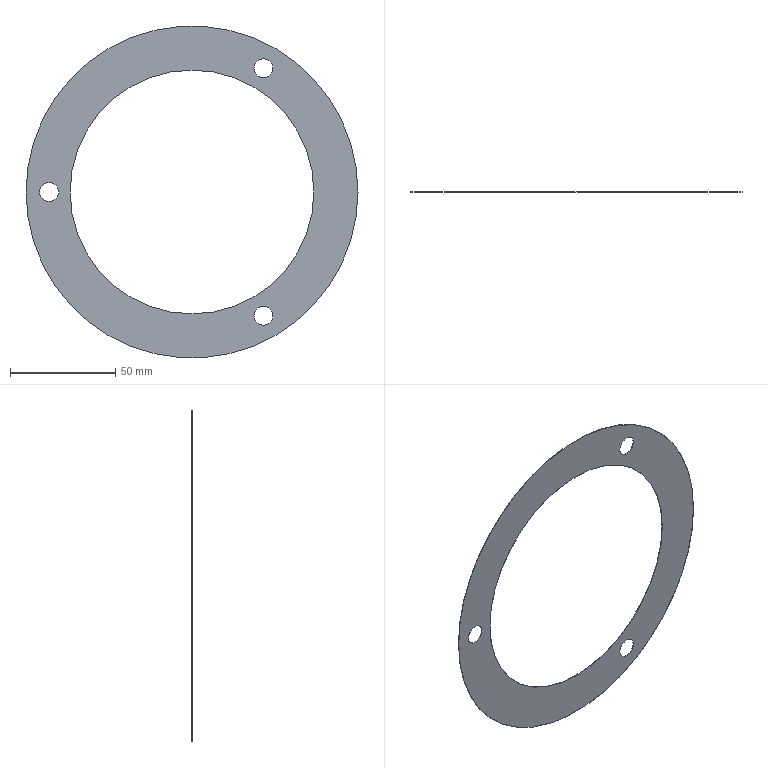Component | SolidWorks | 22-1 | 1 solid | 12 faces | box 158 x 0.2 x 158 mm | volume 1770 mm3 | cylinder 10 | plane 2 | commonest cylinder face diameters 9 x6 116 x2 158 x2
build123d program:
from build123d import *

# Parameters (mm, degrees)
SKETCH1_R           = 79
SKETCH1_R_2         = 58
SKETCH1_R_3         = 4.5
BOSS_EXTRUDE1_DEPTH = 0.2


with BuildPart() as part:
    # Sketch1 → Boss-Extrude1 (new body)
    with BuildSketch(Plane(origin=(0, 0, 0), x_dir=(1, 0, 0), z_dir=(0, 1, 0))):
        with Locations(Location((0, 0, 0), (0, 0, 270))):
            Circle(SKETCH1_R)
        with Locations(Location((0, 0, 0), (0, 0, 270))):
            Circle(SKETCH1_R_2, mode=Mode.SUBTRACT)
        with Locations(Location((0, -68, 0), (0, 0, 270))):
            Circle(SKETCH1_R_3, mode=Mode.SUBTRACT)
        with Locations(Location((-58.89, 34, 0), (0, 0, 270))):
            Circle(SKETCH1_R_3, mode=Mode.SUBTRACT)
        with Locations(Location((58.89, 34, 0), (0, 0, 270))):
            Circle(SKETCH1_R_3, mode=Mode.SUBTRACT)
    extrude(amount=BOSS_EXTRUDE1_DEPTH)


solid = part.part

# Placed as in the assembly
solid = solid.moved(Location((0, 15, 0), (0, -90, 0)))
STEP:
#1=COLOUR_RGB('',0.7922,0.8196,0.9333);
#2=FILL_AREA_STYLE_COLOUR('',#1);
#3=FILL_AREA_STYLE('',(#2));
#4=SURFACE_STYLE_FILL_AREA(#3);
#5=SURFACE_SIDE_STYLE('',(#4));
#6=SURFACE_STYLE_USAGE(.BOTH.,#5);
#7=PRESENTATION_STYLE_ASSIGNMENT((#6));
#8=CARTESIAN_POINT('',(1.516,0.5984,2.318));
#9=VERTEX_POINT('',#8);
#10=CARTESIAN_POINT('',(1.161,0.5984,2.318));
#11=VERTEX_POINT('',#10);
#12=CARTESIAN_POINT('',(1.339,0.5984,2.318));
#13=DIRECTION('',(-0.,1.,0.));
#14=DIRECTION('',(-1.,0.,0.));
#15=AXIS2_PLACEMENT_3D('',#12,#13,#14);
#16=CIRCLE('',#15,0.1772);
#17=EDGE_CURVE('',#9,#11,#16,.T.);
#18=ORIENTED_EDGE('',*,*,#17,.T.);
#19=CARTESIAN_POINT('',(1.161,0.5906,2.318));
#20=VERTEX_POINT('',#19);
#21=CARTESIAN_POINT('',(1.161,0.5984,2.318));
#22=DIRECTION('',(0.,-1.,-0.));
#23=VECTOR('',#22,39.37);
#24=LINE('',#21,#23);
#25=EDGE_CURVE('',#11,#20,#24,.T.);
#26=ORIENTED_EDGE('',*,*,#25,.T.);
#27=CARTESIAN_POINT('',(1.516,0.5906,2.318));
#28=VERTEX_POINT('',#27);
#29=CARTESIAN_POINT('',(1.339,0.5906,2.318));
#30=DIRECTION('',(-0.,1.,0.));
#31=DIRECTION('',(-1.,0.,0.));
#32=AXIS2_PLACEMENT_3D('',#29,#30,#31);
#33=CIRCLE('',#32,0.1772);
#34=EDGE_CURVE('',#28,#20,#33,.T.);
#35=ORIENTED_EDGE('',*,*,#34,.F.);
#36=CARTESIAN_POINT('',(1.516,0.5984,2.318));
#37=DIRECTION('',(0.,-1.,-0.));
#38=VECTOR('',#37,39.37);
#39=LINE('',#36,#38);
#40=EDGE_CURVE('',#9,#28,#39,.T.);
#41=ORIENTED_EDGE('',*,*,#40,.F.);
#42=EDGE_LOOP('',(#18,#26,#35,#41));
#43=FACE_OUTER_BOUND('',#42,.T.);
#44=CARTESIAN_POINT('',(1.339,0.5984,2.318));
#45=DIRECTION('',(0.,-1.,-0.));
#46=DIRECTION('',(1.,0.,-0.));
#47=AXIS2_PLACEMENT_3D('',#44,#45,#46);
#48=CYLINDRICAL_SURFACE('',#47,0.1772);
#49=ADVANCED_FACE('',(#43),#48,.F.);
#50=CARTESIAN_POINT('',(1.516,0.5984,-2.318));
#51=VERTEX_POINT('',#50);
#52=CARTESIAN_POINT('',(1.161,0.5984,-2.318));
#53=VERTEX_POINT('',#52);
#54=CARTESIAN_POINT('',(1.339,0.5984,-2.318));
#55=DIRECTION('',(-0.,1.,0.));
#56=DIRECTION('',(-1.,0.,0.));
#57=AXIS2_PLACEMENT_3D('',#54,#55,#56);
#58=CIRCLE('',#57,0.1772);
#59=EDGE_CURVE('',#51,#53,#58,.T.);
#60=ORIENTED_EDGE('',*,*,#59,.T.);
#61=CARTESIAN_POINT('',(1.161,0.5906,-2.318));
#62=VERTEX_POINT('',#61);
#63=CARTESIAN_POINT('',(1.161,0.5984,-2.318));
#64=DIRECTION('',(0.,-1.,-0.));
#65=VECTOR('',#64,39.37);
#66=LINE('',#63,#65);
#67=EDGE_CURVE('',#53,#62,#66,.T.);
#68=ORIENTED_EDGE('',*,*,#67,.T.);
#69=CARTESIAN_POINT('',(1.516,0.5906,-2.318));
#70=VERTEX_POINT('',#69);
#71=CARTESIAN_POINT('',(1.339,0.5906,-2.318));
#72=DIRECTION('',(-0.,1.,0.));
#73=DIRECTION('',(-1.,0.,0.));
#74=AXIS2_PLACEMENT_3D('',#71,#72,#73);
#75=CIRCLE('',#74,0.1772);
#76=EDGE_CURVE('',#70,#62,#75,.T.);
#77=ORIENTED_EDGE('',*,*,#76,.F.);
#78=CARTESIAN_POINT('',(1.516,0.5984,-2.318));
#79=DIRECTION('',(0.,-1.,-0.));
#80=VECTOR('',#79,39.37);
#81=LINE('',#78,#80);
#82=EDGE_CURVE('',#51,#70,#81,.T.);
#83=ORIENTED_EDGE('',*,*,#82,.F.);
#84=EDGE_LOOP('',(#60,#68,#77,#83));
#85=FACE_OUTER_BOUND('',#84,.T.);
#86=CARTESIAN_POINT('',(1.339,0.5984,-2.318));
#87=DIRECTION('',(0.,-1.,-0.));
#88=DIRECTION('',(1.,0.,-0.));
#89=AXIS2_PLACEMENT_3D('',#86,#87,#88);
#90=CYLINDRICAL_SURFACE('',#89,0.1772);
#91=ADVANCED_FACE('',(#85),#90,.F.);
#92=CARTESIAN_POINT('',(-2.5,0.5984,0.));
#93=VERTEX_POINT('',#92);
#94=CARTESIAN_POINT('',(-2.854,0.5984,0.));
#95=VERTEX_POINT('',#94);
#96=CARTESIAN_POINT('',(-2.677,0.5984,0.));
#97=DIRECTION('',(-0.,1.,0.));
#98=DIRECTION('',(-1.,0.,0.));
#99=AXIS2_PLACEMENT_3D('',#96,#97,#98);
#100=CIRCLE('',#99,0.1772);
#101=EDGE_CURVE('',#93,#95,#100,.T.);
#102=ORIENTED_EDGE('',*,*,#101,.T.);
#103=CARTESIAN_POINT('',(-2.854,0.5906,0.));
#104=VERTEX_POINT('',#103);
#105=CARTESIAN_POINT('',(-2.854,0.5984,0.));
#106=DIRECTION('',(0.,-1.,-0.));
#107=VECTOR('',#106,39.37);
#108=LINE('',#105,#107);
#109=EDGE_CURVE('',#95,#104,#108,.T.);
#110=ORIENTED_EDGE('',*,*,#109,.T.);
#111=CARTESIAN_POINT('',(-2.5,0.5906,0.));
#112=VERTEX_POINT('',#111);
#113=CARTESIAN_POINT('',(-2.677,0.5906,0.));
#114=DIRECTION('',(-0.,1.,0.));
#115=DIRECTION('',(-1.,0.,0.));
#116=AXIS2_PLACEMENT_3D('',#113,#114,#115);
#117=CIRCLE('',#116,0.1772);
#118=EDGE_CURVE('',#112,#104,#117,.T.);
#119=ORIENTED_EDGE('',*,*,#118,.F.);
#120=CARTESIAN_POINT('',(-2.5,0.5984,0.));
#121=DIRECTION('',(0.,-1.,-0.));
#122=VECTOR('',#121,39.37);
#123=LINE('',#120,#122);
#124=EDGE_CURVE('',#93,#112,#123,.T.);
#125=ORIENTED_EDGE('',*,*,#124,.F.);
#126=EDGE_LOOP('',(#102,#110,#119,#125));
#127=FACE_OUTER_BOUND('',#126,.T.);
#128=CARTESIAN_POINT('',(-2.677,0.5984,0.));
#129=DIRECTION('',(0.,-1.,-0.));
#130=DIRECTION('',(1.,0.,-0.));
#131=AXIS2_PLACEMENT_3D('',#128,#129,#130);
#132=CYLINDRICAL_SURFACE('',#131,0.1772);
#133=ADVANCED_FACE('',(#127),#132,.F.);
#134=CARTESIAN_POINT('',(2.283,0.5984,-0.));
#135=VERTEX_POINT('',#134);
#136=CARTESIAN_POINT('',(-2.283,0.5984,0.));
#137=VERTEX_POINT('',#136);
#138=CARTESIAN_POINT('',(0.,0.5984,0.));
#139=DIRECTION('',(-0.,1.,0.));
#140=DIRECTION('',(-1.,-0.,0.));
#141=AXIS2_PLACEMENT_3D('',#138,#139,#140);
#142=CIRCLE('',#141,2.283);
#143=EDGE_CURVE('',#135,#137,#142,.T.);
#144=ORIENTED_EDGE('',*,*,#143,.T.);
#145=CARTESIAN_POINT('',(-2.283,0.5906,0.));
#146=VERTEX_POINT('',#145);
#147=CARTESIAN_POINT('',(-2.283,0.5984,0.));
#148=DIRECTION('',(0.,-1.,-0.));
#149=VECTOR('',#148,39.37);
#150=LINE('',#147,#149);
#151=EDGE_CURVE('',#137,#146,#150,.T.);
#152=ORIENTED_EDGE('',*,*,#151,.T.);
#153=CARTESIAN_POINT('',(2.283,0.5906,-0.));
#154=VERTEX_POINT('',#153);
#155=CARTESIAN_POINT('',(0.,0.5906,0.));
#156=DIRECTION('',(-0.,1.,0.));
#157=DIRECTION('',(-1.,-0.,0.));
#158=AXIS2_PLACEMENT_3D('',#155,#156,#157);
#159=CIRCLE('',#158,2.283);
#160=EDGE_CURVE('',#154,#146,#159,.T.);
#161=ORIENTED_EDGE('',*,*,#160,.F.);
#162=CARTESIAN_POINT('',(2.283,0.5984,-0.));
#163=DIRECTION('',(0.,-1.,-0.));
#164=VECTOR('',#163,39.37);
#165=LINE('',#162,#164);
#166=EDGE_CURVE('',#135,#154,#165,.T.);
#167=ORIENTED_EDGE('',*,*,#166,.F.);
#168=EDGE_LOOP('',(#144,#152,#161,#167));
#169=FACE_OUTER_BOUND('',#168,.T.);
#170=CARTESIAN_POINT('',(0.,0.5984,0.));
#171=DIRECTION('',(0.,-1.,-0.));
#172=DIRECTION('',(1.,0.,-0.));
#173=AXIS2_PLACEMENT_3D('',#170,#171,#172);
#174=CYLINDRICAL_SURFACE('',#173,2.283);
#175=ADVANCED_FACE('',(#169),#174,.F.);
#176=CARTESIAN_POINT('',(-3.11,0.5984,0.));
#177=VERTEX_POINT('',#176);
#178=CARTESIAN_POINT('',(3.11,0.5984,-0.));
#179=VERTEX_POINT('',#178);
#180=CARTESIAN_POINT('',(0.,0.5984,0.));
#181=DIRECTION('',(-0.,1.,0.));
#182=DIRECTION('',(-1.,-0.,0.));
#183=AXIS2_PLACEMENT_3D('',#180,#181,#182);
#184=CIRCLE('',#183,3.11);
#185=EDGE_CURVE('',#177,#179,#184,.T.);
#186=ORIENTED_EDGE('',*,*,#185,.F.);
#187=CARTESIAN_POINT('',(-3.11,0.5906,0.));
#188=VERTEX_POINT('',#187);
#189=CARTESIAN_POINT('',(-3.11,0.5984,0.));
#190=DIRECTION('',(0.,-1.,-0.));
#191=VECTOR('',#190,39.37);
#192=LINE('',#189,#191);
#193=EDGE_CURVE('',#177,#188,#192,.T.);
#194=ORIENTED_EDGE('',*,*,#193,.T.);
#195=CARTESIAN_POINT('',(3.11,0.5906,-0.));
#196=VERTEX_POINT('',#195);
#197=CARTESIAN_POINT('',(0.,0.5906,0.));
#198=DIRECTION('',(-0.,1.,0.));
#199=DIRECTION('',(-1.,-0.,0.));
#200=AXIS2_PLACEMENT_3D('',#197,#198,#199);
#201=CIRCLE('',#200,3.11);
#202=EDGE_CURVE('',#188,#196,#201,.T.);
#203=ORIENTED_EDGE('',*,*,#202,.T.);
#204=CARTESIAN_POINT('',(3.11,0.5984,-0.));
#205=DIRECTION('',(0.,-1.,-0.));
#206=VECTOR('',#205,39.37);
#207=LINE('',#204,#206);
#208=EDGE_CURVE('',#179,#196,#207,.T.);
#209=ORIENTED_EDGE('',*,*,#208,.F.);
#210=EDGE_LOOP('',(#186,#194,#203,#209));
#211=FACE_OUTER_BOUND('',#210,.T.);
#212=CARTESIAN_POINT('',(0.,0.5984,0.));
#213=DIRECTION('',(0.,-1.,-0.));
#214=DIRECTION('',(1.,0.,-0.));
#215=AXIS2_PLACEMENT_3D('',#212,#213,#214);
#216=CYLINDRICAL_SURFACE('',#215,3.11);
#217=ADVANCED_FACE('',(#211),#216,.T.);
#218=ORIENTED_EDGE('',*,*,#59,.F.);
#219=CARTESIAN_POINT('',(1.339,0.5984,-2.318));
#220=DIRECTION('',(-0.,1.,0.));
#221=DIRECTION('',(-1.,0.,0.));
#222=AXIS2_PLACEMENT_3D('',#219,#220,#221);
#223=CIRCLE('',#222,0.1772);
#224=EDGE_CURVE('',#53,#51,#223,.T.);
#225=ORIENTED_EDGE('',*,*,#224,.F.);
#226=EDGE_LOOP('',(#218,#225));
#227=FACE_BOUND('',#226,.T.);
#228=ORIENTED_EDGE('',*,*,#143,.F.);
#229=CARTESIAN_POINT('',(0.,0.5984,0.));
#230=DIRECTION('',(-0.,1.,0.));
#231=DIRECTION('',(-1.,-0.,0.));
#232=AXIS2_PLACEMENT_3D('',#229,#230,#231);
#233=CIRCLE('',#232,2.283);
#234=EDGE_CURVE('',#137,#135,#233,.T.);
#235=ORIENTED_EDGE('',*,*,#234,.F.);
#236=EDGE_LOOP('',(#228,#235));
#237=FACE_BOUND('',#236,.T.);
#238=CARTESIAN_POINT('',(0.,0.5984,0.));
#239=DIRECTION('',(-0.,1.,0.));
#240=DIRECTION('',(-1.,-0.,0.));
#241=AXIS2_PLACEMENT_3D('',#238,#239,#240);
#242=CIRCLE('',#241,3.11);
#243=EDGE_CURVE('',#179,#177,#242,.T.);
#244=ORIENTED_EDGE('',*,*,#243,.T.);
#245=ORIENTED_EDGE('',*,*,#185,.T.);
#246=EDGE_LOOP('',(#244,#245));
#247=FACE_OUTER_BOUND('',#246,.T.);
#248=ORIENTED_EDGE('',*,*,#101,.F.);
#249=CARTESIAN_POINT('',(-2.677,0.5984,0.));
#250=DIRECTION('',(-0.,1.,0.));
#251=DIRECTION('',(-1.,0.,0.));
#252=AXIS2_PLACEMENT_3D('',#249,#250,#251);
#253=CIRCLE('',#252,0.1772);
#254=EDGE_CURVE('',#95,#93,#253,.T.);
#255=ORIENTED_EDGE('',*,*,#254,.F.);
#256=EDGE_LOOP('',(#248,#255));
#257=FACE_BOUND('',#256,.T.);
#258=ORIENTED_EDGE('',*,*,#17,.F.);
#259=CARTESIAN_POINT('',(1.339,0.5984,2.318));
#260=DIRECTION('',(-0.,1.,0.));
#261=DIRECTION('',(-1.,0.,0.));
#262=AXIS2_PLACEMENT_3D('',#259,#260,#261);
#263=CIRCLE('',#262,0.1772);
#264=EDGE_CURVE('',#11,#9,#263,.T.);
#265=ORIENTED_EDGE('',*,*,#264,.F.);
#266=EDGE_LOOP('',(#258,#265));
#267=FACE_BOUND('',#266,.T.);
#268=CARTESIAN_POINT('',(0.,0.5984,0.));
#269=DIRECTION('',(-0.,1.,0.));
#270=DIRECTION('',(-1.,-0.,0.));
#271=AXIS2_PLACEMENT_3D('',#268,#269,#270);
#272=PLANE('',#271);
#273=ADVANCED_FACE('',(#227,#237,#247,#257,#267),#272,.T.);
#274=CARTESIAN_POINT('',(0.,0.5906,0.));
#275=DIRECTION('',(-0.,1.,0.));
#276=DIRECTION('',(-1.,-0.,0.));
#277=AXIS2_PLACEMENT_3D('',#274,#275,#276);
#278=CIRCLE('',#277,3.11);
#279=EDGE_CURVE('',#196,#188,#278,.T.);
#280=ORIENTED_EDGE('',*,*,#279,.F.);
#281=ORIENTED_EDGE('',*,*,#202,.F.);
#282=EDGE_LOOP('',(#280,#281));
#283=FACE_OUTER_BOUND('',#282,.T.);
#284=ORIENTED_EDGE('',*,*,#160,.T.);
#285=CARTESIAN_POINT('',(0.,0.5906,0.));
#286=DIRECTION('',(-0.,1.,0.));
#287=DIRECTION('',(-1.,-0.,0.));
#288=AXIS2_PLACEMENT_3D('',#285,#286,#287);
#289=CIRCLE('',#288,2.283);
#290=EDGE_CURVE('',#146,#154,#289,.T.);
#291=ORIENTED_EDGE('',*,*,#290,.T.);
#292=EDGE_LOOP('',(#284,#291));
#293=FACE_BOUND('',#292,.T.);
#294=ORIENTED_EDGE('',*,*,#118,.T.);
#295=CARTESIAN_POINT('',(-2.677,0.5906,0.));
#296=DIRECTION('',(-0.,1.,0.));
#297=DIRECTION('',(-1.,0.,0.));
#298=AXIS2_PLACEMENT_3D('',#295,#296,#297);
#299=CIRCLE('',#298,0.1772);
#300=EDGE_CURVE('',#104,#112,#299,.T.);
#301=ORIENTED_EDGE('',*,*,#300,.T.);
#302=EDGE_LOOP('',(#294,#301));
#303=FACE_BOUND('',#302,.T.);
#304=ORIENTED_EDGE('',*,*,#76,.T.);
#305=CARTESIAN_POINT('',(1.339,0.5906,-2.318));
#306=DIRECTION('',(-0.,1.,0.));
#307=DIRECTION('',(-1.,0.,0.));
#308=AXIS2_PLACEMENT_3D('',#305,#306,#307);
#309=CIRCLE('',#308,0.1772);
#310=EDGE_CURVE('',#62,#70,#309,.T.);
#311=ORIENTED_EDGE('',*,*,#310,.T.);
#312=EDGE_LOOP('',(#304,#311));
#313=FACE_BOUND('',#312,.T.);
#314=ORIENTED_EDGE('',*,*,#34,.T.);
#315=CARTESIAN_POINT('',(1.339,0.5906,2.318));
#316=DIRECTION('',(-0.,1.,0.));
#317=DIRECTION('',(-1.,0.,0.));
#318=AXIS2_PLACEMENT_3D('',#315,#316,#317);
#319=CIRCLE('',#318,0.1772);
#320=EDGE_CURVE('',#20,#28,#319,.T.);
#321=ORIENTED_EDGE('',*,*,#320,.T.);
#322=EDGE_LOOP('',(#314,#321));
#323=FACE_BOUND('',#322,.T.);
#324=CARTESIAN_POINT('',(0.,0.5906,0.));
#325=DIRECTION('',(-0.,1.,0.));
#326=DIRECTION('',(-1.,-0.,0.));
#327=AXIS2_PLACEMENT_3D('',#324,#325,#326);
#328=PLANE('',#327);
#329=ADVANCED_FACE('',(#283,#293,#303,#313,#323),#328,.F.);
#330=ORIENTED_EDGE('',*,*,#193,.F.);
#331=ORIENTED_EDGE('',*,*,#243,.F.);
#332=ORIENTED_EDGE('',*,*,#208,.T.);
#333=ORIENTED_EDGE('',*,*,#279,.T.);
#334=EDGE_LOOP('',(#330,#331,#332,#333));
#335=FACE_OUTER_BOUND('',#334,.T.);
#336=CARTESIAN_POINT('',(0.,0.5984,0.));
#337=DIRECTION('',(0.,-1.,-0.));
#338=DIRECTION('',(1.,0.,-0.));
#339=AXIS2_PLACEMENT_3D('',#336,#337,#338);
#340=CYLINDRICAL_SURFACE('',#339,3.11);
#341=ADVANCED_FACE('',(#335),#340,.T.);
#342=ORIENTED_EDGE('',*,*,#151,.F.);
#343=ORIENTED_EDGE('',*,*,#234,.T.);
#344=ORIENTED_EDGE('',*,*,#166,.T.);
#345=ORIENTED_EDGE('',*,*,#290,.F.);
#346=EDGE_LOOP('',(#342,#343,#344,#345));
#347=FACE_OUTER_BOUND('',#346,.T.);
#348=CARTESIAN_POINT('',(0.,0.5984,0.));
#349=DIRECTION('',(0.,-1.,-0.));
#350=DIRECTION('',(1.,0.,-0.));
#351=AXIS2_PLACEMENT_3D('',#348,#349,#350);
#352=CYLINDRICAL_SURFACE('',#351,2.283);
#353=ADVANCED_FACE('',(#347),#352,.F.);
#354=ORIENTED_EDGE('',*,*,#109,.F.);
#355=ORIENTED_EDGE('',*,*,#254,.T.);
#356=ORIENTED_EDGE('',*,*,#124,.T.);
#357=ORIENTED_EDGE('',*,*,#300,.F.);
#358=EDGE_LOOP('',(#354,#355,#356,#357));
#359=FACE_OUTER_BOUND('',#358,.T.);
#360=CARTESIAN_POINT('',(-2.677,0.5984,0.));
#361=DIRECTION('',(0.,-1.,-0.));
#362=DIRECTION('',(1.,0.,-0.));
#363=AXIS2_PLACEMENT_3D('',#360,#361,#362);
#364=CYLINDRICAL_SURFACE('',#363,0.1772);
#365=ADVANCED_FACE('',(#359),#364,.F.);
#366=ORIENTED_EDGE('',*,*,#67,.F.);
#367=ORIENTED_EDGE('',*,*,#224,.T.);
#368=ORIENTED_EDGE('',*,*,#82,.T.);
#369=ORIENTED_EDGE('',*,*,#310,.F.);
#370=EDGE_LOOP('',(#366,#367,#368,#369));
#371=FACE_OUTER_BOUND('',#370,.T.);
#372=CARTESIAN_POINT('',(1.339,0.5984,-2.318));
#373=DIRECTION('',(0.,-1.,-0.));
#374=DIRECTION('',(1.,0.,-0.));
#375=AXIS2_PLACEMENT_3D('',#372,#373,#374);
#376=CYLINDRICAL_SURFACE('',#375,0.1772);
#377=ADVANCED_FACE('',(#371),#376,.F.);
#378=ORIENTED_EDGE('',*,*,#25,.F.);
#379=ORIENTED_EDGE('',*,*,#264,.T.);
#380=ORIENTED_EDGE('',*,*,#40,.T.);
#381=ORIENTED_EDGE('',*,*,#320,.F.);
#382=EDGE_LOOP('',(#378,#379,#380,#381));
#383=FACE_OUTER_BOUND('',#382,.T.);
#384=CARTESIAN_POINT('',(1.339,0.5984,2.318));
#385=DIRECTION('',(0.,-1.,-0.));
#386=DIRECTION('',(1.,0.,-0.));
#387=AXIS2_PLACEMENT_3D('',#384,#385,#386);
#388=CYLINDRICAL_SURFACE('',#387,0.1772);
#389=ADVANCED_FACE('',(#383),#388,.F.);
#390=CLOSED_SHELL('',(#49,#91,#133,#175,#217,#273,#329,#341,#353,#365,#377,#389));
#391=MANIFOLD_SOLID_BREP('',#390);
#392=STYLED_ITEM('',(#7),#391);
#393=PRESENTATION_LAYER_ASSIGNMENT('','',(#392));
#394=CARTESIAN_POINT('',(0.,0.,0.));
#395=DIRECTION('',(0.,0.,1.));
#396=DIRECTION('',(1.,0.,0.));
#397=AXIS2_PLACEMENT_3D('',#394,#395,#396);
#398=(LENGTH_UNIT()NAMED_UNIT(*)SI_UNIT($,.METRE.));
#399=LENGTH_MEASURE_WITH_UNIT(LENGTH_MEASURE(0.0254),#398);
#400=DIMENSIONAL_EXPONENTS(1.,0.,0.,0.,0.,0.,0.);
#401=(CONVERSION_BASED_UNIT('',#399)LENGTH_UNIT()NAMED_UNIT(#400));
#402=UNCERTAINTY_MEASURE_WITH_UNIT(LENGTH_MEASURE(0.00001),#401,'','');
#403=(NAMED_UNIT(*)PLANE_ANGLE_UNIT()SI_UNIT($,.RADIAN.));
#404=(NAMED_UNIT(*)SI_UNIT($,.STERADIAN.)SOLID_ANGLE_UNIT());
#405=(GEOMETRIC_REPRESENTATION_CONTEXT(3)GLOBAL_UNCERTAINTY_ASSIGNED_CONTEXT((#402))GLOBAL_UNIT_ASSIGNED_CONTEXT((#401,#403,#404))REPRESENTATION_CONTEXT('',''));
#406=ADVANCED_BREP_SHAPE_REPRESENTATION('',(#391,#397),#405);
#407=(LENGTH_UNIT()NAMED_UNIT(*)SI_UNIT($,.METRE.));
#408=LENGTH_MEASURE_WITH_UNIT(LENGTH_MEASURE(0.0254),#407);
#409=DIMENSIONAL_EXPONENTS(1.,0.,0.,0.,0.,0.,0.);
#410=(CONVERSION_BASED_UNIT('',#408)LENGTH_UNIT()NAMED_UNIT(#409));
#411=UNCERTAINTY_MEASURE_WITH_UNIT(LENGTH_MEASURE(0.00001),#410,'','');
#412=(NAMED_UNIT(*)PLANE_ANGLE_UNIT()SI_UNIT($,.RADIAN.));
#413=(NAMED_UNIT(*)SI_UNIT($,.STERADIAN.)SOLID_ANGLE_UNIT());
#414=(GEOMETRIC_REPRESENTATION_CONTEXT(3)GLOBAL_UNCERTAINTY_ASSIGNED_CONTEXT((#411))GLOBAL_UNIT_ASSIGNED_CONTEXT((#410,#412,#413))REPRESENTATION_CONTEXT('',''));
#415=MECHANICAL_DESIGN_GEOMETRIC_PRESENTATION_REPRESENTATION('',(#392),#414);